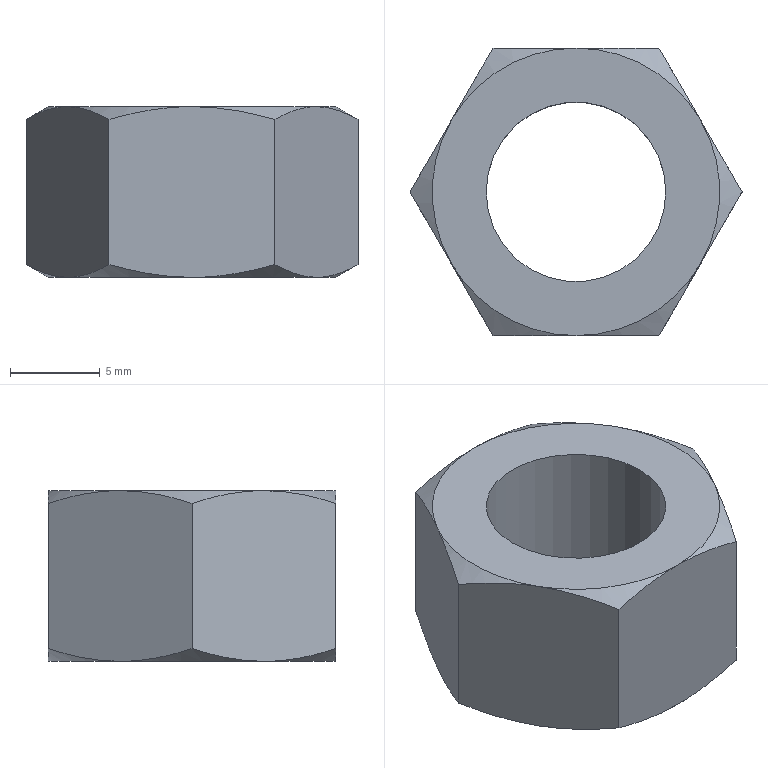Component | NX | NUT_M10 | 1 solid | 21 faces | volume 1351 mm3 | cone 12 | plane 8 | cylinder 1 | commonest cylinder face diameters 10 x1